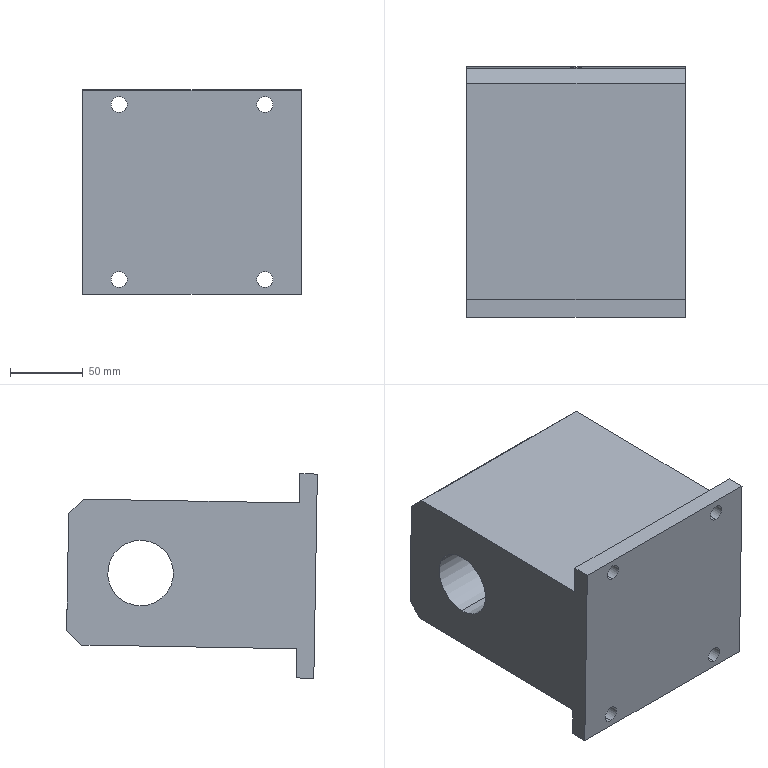Component | SolidWorks | Tailstock-1 | 1 solid | 24 faces | box 150 x 171.89 x 140.19 mm | volume 2362487 mm3 | cylinder 12 | plane 12 | commonest cylinder face diameters 11 x8 8 x2 45 x2
build123d program:
from build123d import *

# Parameters (mm, degrees)
SKETCH1_R           = 22.5
BOSS_EXTRUDE1_DEPTH = 75
CHAMFER1_SIZE       = 10
SKETCH2_R           = 5.5
CUT_EXTRUDE1_DEPTH  = 189.385
SKETCH3_R           = 4
CUT_EXTRUDE2_DEPTH  = 30


with BuildPart() as part:
    # Sketch1 → Boss-Extrude1 (new, symmetric)
    with BuildSketch(Plane.XY):
        Polygon((70, 0), (-70, 0), (-70, 12), (-50, 12), (-50, 170), (50, 170), (50, 12), (70, 12), align=None)
        with Locations((0, 120)):
            Circle(SKETCH1_R, mode=Mode.SUBTRACT)
    extrude(amount=BOSS_EXTRUDE1_DEPTH, both=True)

    # Chamfer1
    chamfer1_edges = [part.edges().sort_by_distance(p)[0] for p in [
        (-50, 170, 0),
        (50, 170, 0),
    ]]
    chamfer(chamfer1_edges, length=CHAMFER1_SIZE)

    # Sketch2 → Cut-Extrude1 (cut, through all)
    with BuildSketch(Plane(origin=(0, 12, 0), x_dir=(1, 0, 0), z_dir=(0, 1, 0))):
        with Locations(Location((-60, 50, 0), (0, 0, 180))):
            Circle(SKETCH2_R)
        with Locations((60, 50)):
            Circle(SKETCH2_R)
        with Locations(Location((60, -50, 0), (0, 0, 180))):
            Circle(SKETCH2_R)
        with Locations((-60, -50)):
            Circle(SKETCH2_R)
    extrude(amount=-CUT_EXTRUDE1_DEPTH, mode=Mode.SUBTRACT)

    # Sketch3 → Cut-Extrude2 (cut)
    with BuildSketch(Plane(origin=(0, 170, 0), x_dir=(1, 0, 0), z_dir=(0, 1, 0))):
        with Locations(Location((0, 0, 0), (0, 0, 270))):
            Circle(SKETCH3_R)
    extrude(amount=-CUT_EXTRUDE2_DEPTH, mode=Mode.SUBTRACT)


solid = part.part

# Placed as in the assembly
solid = solid.moved(Location((592.004, 1179.724, 685.022), (1, 90, 0)))
STEP:
#1=CARTESIAN_POINT('',(23.15,52.055,27.067));
#2=VERTEX_POINT('',#1);
#3=CARTESIAN_POINT('',(23.465,52.055,27.067));
#4=VERTEX_POINT('',#3);
#5=CARTESIAN_POINT('',(23.15,52.055,27.067));
#6=CARTESIAN_POINT('',(23.15,52.055,27.057));
#7=CARTESIAN_POINT('',(23.151,52.055,27.047));
#8=CARTESIAN_POINT('',(23.155,52.055,27.026));
#9=CARTESIAN_POINT('',(23.158,52.055,27.016));
#10=CARTESIAN_POINT('',(23.166,52.054,26.997));
#11=CARTESIAN_POINT('',(23.171,52.053,26.988));
#12=CARTESIAN_POINT('',(23.182,52.052,26.971));
#13=CARTESIAN_POINT('',(23.189,52.051,26.963));
#14=CARTESIAN_POINT('',(23.203,52.049,26.949));
#15=CARTESIAN_POINT('',(23.211,52.049,26.942));
#16=CARTESIAN_POINT('',(23.228,52.047,26.93));
#17=CARTESIAN_POINT('',(23.237,52.046,26.926));
#18=CARTESIAN_POINT('',(23.256,52.045,26.918));
#19=CARTESIAN_POINT('',(23.266,52.045,26.915));
#20=CARTESIAN_POINT('',(23.287,52.044,26.911));
#21=CARTESIAN_POINT('',(23.297,52.044,26.91));
#22=CARTESIAN_POINT('',(23.317,52.044,26.91));
#23=CARTESIAN_POINT('',(23.328,52.044,26.911));
#24=CARTESIAN_POINT('',(23.348,52.045,26.915));
#25=CARTESIAN_POINT('',(23.358,52.045,26.918));
#26=CARTESIAN_POINT('',(23.377,52.046,26.926));
#27=CARTESIAN_POINT('',(23.386,52.047,26.93));
#28=CARTESIAN_POINT('',(23.403,52.049,26.942));
#29=CARTESIAN_POINT('',(23.411,52.049,26.948));
#30=CARTESIAN_POINT('',(23.426,52.051,26.963));
#31=CARTESIAN_POINT('',(23.432,52.052,26.971));
#32=CARTESIAN_POINT('',(23.444,52.053,26.988));
#33=CARTESIAN_POINT('',(23.449,52.054,26.997));
#34=CARTESIAN_POINT('',(23.457,52.055,27.016));
#35=CARTESIAN_POINT('',(23.46,52.055,27.026));
#36=CARTESIAN_POINT('',(23.464,52.055,27.047));
#37=CARTESIAN_POINT('',(23.465,52.055,27.057));
#38=CARTESIAN_POINT('',(23.465,52.055,27.067));
#39=B_SPLINE_CURVE_WITH_KNOTS('',3,(#5,#6,#7,#8,#9,#10,#11,#12,#13,#14,#15,#16,#17,#18,#19,#20,#21,#22,#23,#24,#25,#26,#27,#28,#29,#30,#31,#32,#33,#34,#35,#36,#37,#38),.UNSPECIFIED.,.F.,.F.,(4,2,2,2,2,2,2,2,2,2,2,2,2,2,2,2,4),(0.,0.0007832,0.001566,0.00235,0.003133,0.003916,0.004699,0.005482,0.006265,0.007049,0.007832,0.008615,0.009398,0.01018,0.01096,0.01175,0.01253),.UNSPECIFIED.);
#40=EDGE_CURVE('',#2,#4,#39,.T.);
#41=ORIENTED_EDGE('',*,*,#40,.T.);
#42=CARTESIAN_POINT('',(23.465,53.138,27.086));
#43=VERTEX_POINT('',#42);
#44=CARTESIAN_POINT('',(23.465,51.957,27.066));
#45=DIRECTION('',(-0.,0.9998,0.01745));
#46=VECTOR('',#45,39.37);
#47=LINE('',#44,#46);
#48=EDGE_CURVE('',#4,#43,#47,.T.);
#49=ORIENTED_EDGE('',*,*,#48,.T.);
#50=CARTESIAN_POINT('',(23.15,53.138,27.086));
#51=VERTEX_POINT('',#50);
#52=CARTESIAN_POINT('',(23.307,53.138,27.086));
#53=DIRECTION('',(-0.,0.9998,0.01745));
#54=DIRECTION('',(-1.,0.,0.));
#55=AXIS2_PLACEMENT_3D('',#52,#53,#54);
#56=CIRCLE('',#55,0.1575);
#57=EDGE_CURVE('',#43,#51,#56,.T.);
#58=ORIENTED_EDGE('',*,*,#57,.T.);
#59=CARTESIAN_POINT('',(23.15,51.957,27.066));
#60=DIRECTION('',(-0.,0.9998,0.01745));
#61=VECTOR('',#60,39.37);
#62=LINE('',#59,#61);
#63=EDGE_CURVE('',#2,#51,#62,.T.);
#64=ORIENTED_EDGE('',*,*,#63,.F.);
#65=EDGE_LOOP('',(#41,#49,#58,#64));
#66=FACE_OUTER_BOUND('',#65,.T.);
#67=CARTESIAN_POINT('',(23.307,51.957,27.066));
#68=DIRECTION('',(-0.,0.9998,0.01745));
#69=DIRECTION('',(-1.,0.,0.));
#70=AXIS2_PLACEMENT_3D('',#67,#68,#69);
#71=CYLINDRICAL_SURFACE('',#70,0.1575);
#72=ADVANCED_FACE('',(#66),#71,.F.);
#73=CARTESIAN_POINT('',(21.339,46.483,24.824));
#74=VERTEX_POINT('',#73);
#75=CARTESIAN_POINT('',(21.339,46.491,24.391));
#76=VERTEX_POINT('',#75);
#77=CARTESIAN_POINT('',(21.339,46.487,24.608));
#78=DIRECTION('',(-0.,0.9998,0.01745));
#79=DIRECTION('',(0.,-0.01745,0.9998));
#80=AXIS2_PLACEMENT_3D('',#77,#78,#79);
#81=CIRCLE('',#80,0.2165);
#82=EDGE_CURVE('',#74,#76,#81,.T.);
#83=ORIENTED_EDGE('',*,*,#82,.F.);
#84=CARTESIAN_POINT('',(21.339,46.956,24.832));
#85=VERTEX_POINT('',#84);
#86=CARTESIAN_POINT('',(21.339,46.483,24.824));
#87=DIRECTION('',(-0.,0.9998,0.01745));
#88=VECTOR('',#87,39.37);
#89=LINE('',#86,#88);
#90=EDGE_CURVE('',#74,#85,#89,.T.);
#91=ORIENTED_EDGE('',*,*,#90,.T.);
#92=CARTESIAN_POINT('',(21.339,46.963,24.399));
#93=VERTEX_POINT('',#92);
#94=CARTESIAN_POINT('',(21.339,46.959,24.616));
#95=DIRECTION('',(-0.,0.9998,0.01745));
#96=DIRECTION('',(0.,-0.01745,0.9998));
#97=AXIS2_PLACEMENT_3D('',#94,#95,#96);
#98=CIRCLE('',#97,0.2165);
#99=EDGE_CURVE('',#85,#93,#98,.T.);
#100=ORIENTED_EDGE('',*,*,#99,.T.);
#101=CARTESIAN_POINT('',(21.339,46.491,24.391));
#102=DIRECTION('',(-0.,0.9998,0.01745));
#103=VECTOR('',#102,39.37);
#104=LINE('',#101,#103);
#105=EDGE_CURVE('',#76,#93,#104,.T.);
#106=ORIENTED_EDGE('',*,*,#105,.F.);
#107=EDGE_LOOP('',(#83,#91,#100,#106));
#108=FACE_OUTER_BOUND('',#107,.T.);
#109=CARTESIAN_POINT('',(21.339,46.487,24.608));
#110=DIRECTION('',(-0.,0.9998,0.01745));
#111=DIRECTION('',(0.,0.01745,-0.9998));
#112=AXIS2_PLACEMENT_3D('',#109,#110,#111);
#113=CYLINDRICAL_SURFACE('',#112,0.2165);
#114=ADVANCED_FACE('',(#108),#113,.F.);
#115=CARTESIAN_POINT('',(21.339,46.401,29.548));
#116=VERTEX_POINT('',#115);
#117=CARTESIAN_POINT('',(21.339,46.408,29.115));
#118=VERTEX_POINT('',#117);
#119=CARTESIAN_POINT('',(21.339,46.405,29.331));
#120=DIRECTION('',(-0.,0.9998,0.01745));
#121=DIRECTION('',(0.,0.01745,-0.9998));
#122=AXIS2_PLACEMENT_3D('',#119,#120,#121);
#123=CIRCLE('',#122,0.2165);
#124=EDGE_CURVE('',#116,#118,#123,.T.);
#125=ORIENTED_EDGE('',*,*,#124,.F.);
#126=CARTESIAN_POINT('',(21.339,46.873,29.556));
#127=VERTEX_POINT('',#126);
#128=CARTESIAN_POINT('',(21.339,46.401,29.548));
#129=DIRECTION('',(-0.,0.9998,0.01745));
#130=VECTOR('',#129,39.37);
#131=LINE('',#128,#130);
#132=EDGE_CURVE('',#116,#127,#131,.T.);
#133=ORIENTED_EDGE('',*,*,#132,.T.);
#134=CARTESIAN_POINT('',(21.339,46.881,29.123));
#135=VERTEX_POINT('',#134);
#136=CARTESIAN_POINT('',(21.339,46.877,29.339));
#137=DIRECTION('',(-0.,0.9998,0.01745));
#138=DIRECTION('',(0.,0.01745,-0.9998));
#139=AXIS2_PLACEMENT_3D('',#136,#137,#138);
#140=CIRCLE('',#139,0.2165);
#141=EDGE_CURVE('',#127,#135,#140,.T.);
#142=ORIENTED_EDGE('',*,*,#141,.T.);
#143=CARTESIAN_POINT('',(21.339,46.408,29.115));
#144=DIRECTION('',(-0.,0.9998,0.01745));
#145=VECTOR('',#144,39.37);
#146=LINE('',#143,#145);
#147=EDGE_CURVE('',#118,#135,#146,.T.);
#148=ORIENTED_EDGE('',*,*,#147,.F.);
#149=EDGE_LOOP('',(#125,#133,#142,#148));
#150=FACE_OUTER_BOUND('',#149,.T.);
#151=CARTESIAN_POINT('',(21.339,46.405,29.331));
#152=DIRECTION('',(-0.,0.9998,0.01745));
#153=DIRECTION('',(0.,0.01745,-0.9998));
#154=AXIS2_PLACEMENT_3D('',#151,#152,#153);
#155=CYLINDRICAL_SURFACE('',#154,0.2165);
#156=ADVANCED_FACE('',(#150),#155,.F.);
#157=CARTESIAN_POINT('',(25.276,46.401,29.548));
#158=VERTEX_POINT('',#157);
#159=CARTESIAN_POINT('',(25.276,46.408,29.115));
#160=VERTEX_POINT('',#159);
#161=CARTESIAN_POINT('',(25.276,46.405,29.331));
#162=DIRECTION('',(-0.,0.9998,0.01745));
#163=DIRECTION('',(0.,-0.01745,0.9998));
#164=AXIS2_PLACEMENT_3D('',#161,#162,#163);
#165=CIRCLE('',#164,0.2165);
#166=EDGE_CURVE('',#158,#160,#165,.T.);
#167=ORIENTED_EDGE('',*,*,#166,.F.);
#168=CARTESIAN_POINT('',(25.276,46.873,29.556));
#169=VERTEX_POINT('',#168);
#170=CARTESIAN_POINT('',(25.276,46.401,29.548));
#171=DIRECTION('',(-0.,0.9998,0.01745));
#172=VECTOR('',#171,39.37);
#173=LINE('',#170,#172);
#174=EDGE_CURVE('',#158,#169,#173,.T.);
#175=ORIENTED_EDGE('',*,*,#174,.T.);
#176=CARTESIAN_POINT('',(25.276,46.881,29.123));
#177=VERTEX_POINT('',#176);
#178=CARTESIAN_POINT('',(25.276,46.877,29.339));
#179=DIRECTION('',(-0.,0.9998,0.01745));
#180=DIRECTION('',(0.,-0.01745,0.9998));
#181=AXIS2_PLACEMENT_3D('',#178,#179,#180);
#182=CIRCLE('',#181,0.2165);
#183=EDGE_CURVE('',#169,#177,#182,.T.);
#184=ORIENTED_EDGE('',*,*,#183,.T.);
#185=CARTESIAN_POINT('',(25.276,46.408,29.115));
#186=DIRECTION('',(-0.,0.9998,0.01745));
#187=VECTOR('',#186,39.37);
#188=LINE('',#185,#187);
#189=EDGE_CURVE('',#160,#177,#188,.T.);
#190=ORIENTED_EDGE('',*,*,#189,.F.);
#191=EDGE_LOOP('',(#167,#175,#184,#190));
#192=FACE_OUTER_BOUND('',#191,.T.);
#193=CARTESIAN_POINT('',(25.276,46.405,29.331));
#194=DIRECTION('',(-0.,0.9998,0.01745));
#195=DIRECTION('',(0.,0.01745,-0.9998));
#196=AXIS2_PLACEMENT_3D('',#193,#194,#195);
#197=CYLINDRICAL_SURFACE('',#196,0.2165);
#198=ADVANCED_FACE('',(#192),#197,.F.);
#199=CARTESIAN_POINT('',(25.276,46.483,24.824));
#200=VERTEX_POINT('',#199);
#201=CARTESIAN_POINT('',(25.276,46.491,24.391));
#202=VERTEX_POINT('',#201);
#203=CARTESIAN_POINT('',(25.276,46.487,24.608));
#204=DIRECTION('',(-0.,0.9998,0.01745));
#205=DIRECTION('',(0.,0.01745,-0.9998));
#206=AXIS2_PLACEMENT_3D('',#203,#204,#205);
#207=CIRCLE('',#206,0.2165);
#208=EDGE_CURVE('',#200,#202,#207,.T.);
#209=ORIENTED_EDGE('',*,*,#208,.F.);
#210=CARTESIAN_POINT('',(25.276,46.956,24.832));
#211=VERTEX_POINT('',#210);
#212=CARTESIAN_POINT('',(25.276,46.483,24.824));
#213=DIRECTION('',(-0.,0.9998,0.01745));
#214=VECTOR('',#213,39.37);
#215=LINE('',#212,#214);
#216=EDGE_CURVE('',#200,#211,#215,.T.);
#217=ORIENTED_EDGE('',*,*,#216,.T.);
#218=CARTESIAN_POINT('',(25.276,46.963,24.399));
#219=VERTEX_POINT('',#218);
#220=CARTESIAN_POINT('',(25.276,46.959,24.616));
#221=DIRECTION('',(-0.,0.9998,0.01745));
#222=DIRECTION('',(0.,0.01745,-0.9998));
#223=AXIS2_PLACEMENT_3D('',#220,#221,#222);
#224=CIRCLE('',#223,0.2165);
#225=EDGE_CURVE('',#211,#219,#224,.T.);
#226=ORIENTED_EDGE('',*,*,#225,.T.);
#227=CARTESIAN_POINT('',(25.276,46.491,24.391));
#228=DIRECTION('',(-0.,0.9998,0.01745));
#229=VECTOR('',#228,39.37);
#230=LINE('',#227,#229);
#231=EDGE_CURVE('',#202,#219,#230,.T.);
#232=ORIENTED_EDGE('',*,*,#231,.F.);
#233=EDGE_LOOP('',(#209,#217,#226,#232));
#234=FACE_OUTER_BOUND('',#233,.T.);
#235=CARTESIAN_POINT('',(25.276,46.487,24.608));
#236=DIRECTION('',(-0.,0.9998,0.01745));
#237=DIRECTION('',(0.,0.01745,-0.9998));
#238=AXIS2_PLACEMENT_3D('',#235,#236,#237);
#239=CYLINDRICAL_SURFACE('',#238,0.2165);
#240=ADVANCED_FACE('',(#234),#239,.F.);
#241=CARTESIAN_POINT('',(20.354,51.185,26.166));
#242=VERTEX_POINT('',#241);
#243=CARTESIAN_POINT('',(20.354,51.154,27.938));
#244=VERTEX_POINT('',#243);
#245=CARTESIAN_POINT('',(20.354,51.17,27.052));
#246=DIRECTION('',(-1.,-0.,-0.));
#247=DIRECTION('',(0.,-0.01745,0.9998));
#248=AXIS2_PLACEMENT_3D('',#245,#246,#247);
#249=CIRCLE('',#248,0.8858);
#250=EDGE_CURVE('',#242,#244,#249,.T.);
#251=ORIENTED_EDGE('',*,*,#250,.T.);
#252=CARTESIAN_POINT('',(26.26,51.154,27.938));
#253=VERTEX_POINT('',#252);
#254=CARTESIAN_POINT('',(20.354,51.154,27.938));
#255=DIRECTION('',(1.,0.,0.));
#256=VECTOR('',#255,39.37);
#257=LINE('',#254,#256);
#258=EDGE_CURVE('',#244,#253,#257,.T.);
#259=ORIENTED_EDGE('',*,*,#258,.T.);
#260=CARTESIAN_POINT('',(26.26,51.185,26.166));
#261=VERTEX_POINT('',#260);
#262=CARTESIAN_POINT('',(26.26,51.17,27.052));
#263=DIRECTION('',(-1.,-0.,-0.));
#264=DIRECTION('',(0.,-0.01745,0.9998));
#265=AXIS2_PLACEMENT_3D('',#262,#263,#264);
#266=CIRCLE('',#265,0.8858);
#267=EDGE_CURVE('',#261,#253,#266,.T.);
#268=ORIENTED_EDGE('',*,*,#267,.F.);
#269=CARTESIAN_POINT('',(20.354,51.185,26.166));
#270=DIRECTION('',(1.,0.,0.));
#271=VECTOR('',#270,39.37);
#272=LINE('',#269,#271);
#273=EDGE_CURVE('',#242,#261,#272,.T.);
#274=ORIENTED_EDGE('',*,*,#273,.F.);
#275=EDGE_LOOP('',(#251,#259,#268,#274));
#276=FACE_OUTER_BOUND('',#275,.T.);
#277=CARTESIAN_POINT('',(20.354,51.17,27.052));
#278=DIRECTION('',(1.,0.,0.));
#279=DIRECTION('',(0.,0.01745,-0.9998));
#280=AXIS2_PLACEMENT_3D('',#277,#278,#279);
#281=CYLINDRICAL_SURFACE('',#280,0.8858);
#282=ADVANCED_FACE('',(#276),#281,.F.);
#283=CARTESIAN_POINT('',(20.354,53.11,28.661));
#284=VERTEX_POINT('',#283);
#285=CARTESIAN_POINT('',(20.354,53.165,25.512));
#286=VERTEX_POINT('',#285);
#287=CARTESIAN_POINT('',(20.354,53.172,25.118));
#288=DIRECTION('',(0.,0.01745,-0.9998));
#289=VECTOR('',#288,39.37);
#290=LINE('',#287,#289);
#291=EDGE_CURVE('',#284,#286,#290,.T.);
#292=ORIENTED_EDGE('',*,*,#291,.T.);
#293=CARTESIAN_POINT('',(20.354,52.778,25.111));
#294=VERTEX_POINT('',#293);
#295=CARTESIAN_POINT('',(20.354,52.778,25.111));
#296=DIRECTION('',(0.,-0.6947,-0.7193));
#297=VECTOR('',#296,39.37);
#298=LINE('',#295,#297);
#299=EDGE_CURVE('',#286,#294,#298,.T.);
#300=ORIENTED_EDGE('',*,*,#299,.T.);
#301=CARTESIAN_POINT('',(20.354,46.953,25.009));
#302=VERTEX_POINT('',#301);
#303=CARTESIAN_POINT('',(20.354,46.953,25.009));
#304=DIRECTION('',(0.,-0.9998,-0.01745));
#305=VECTOR('',#304,39.37);
#306=LINE('',#303,#305);
#307=EDGE_CURVE('',#294,#302,#306,.T.);
#308=ORIENTED_EDGE('',*,*,#307,.T.);
#309=CARTESIAN_POINT('',(20.354,46.966,24.222));
#310=VERTEX_POINT('',#309);
#311=CARTESIAN_POINT('',(20.354,46.966,24.222));
#312=DIRECTION('',(-0.,0.01745,-0.9998));
#313=VECTOR('',#312,39.37);
#314=LINE('',#311,#313);
#315=EDGE_CURVE('',#302,#310,#314,.T.);
#316=ORIENTED_EDGE('',*,*,#315,.T.);
#317=CARTESIAN_POINT('',(20.354,46.494,24.214));
#318=VERTEX_POINT('',#317);
#319=CARTESIAN_POINT('',(20.354,46.494,24.214));
#320=DIRECTION('',(0.,-0.9998,-0.01745));
#321=VECTOR('',#320,39.37);
#322=LINE('',#319,#321);
#323=EDGE_CURVE('',#310,#318,#322,.T.);
#324=ORIENTED_EDGE('',*,*,#323,.T.);
#325=CARTESIAN_POINT('',(20.354,46.398,29.725));
#326=VERTEX_POINT('',#325);
#327=CARTESIAN_POINT('',(20.354,46.398,29.725));
#328=DIRECTION('',(0.,-0.01745,0.9998));
#329=VECTOR('',#328,39.37);
#330=LINE('',#327,#329);
#331=EDGE_CURVE('',#318,#326,#330,.T.);
#332=ORIENTED_EDGE('',*,*,#331,.T.);
#333=CARTESIAN_POINT('',(20.354,46.87,29.733));
#334=VERTEX_POINT('',#333);
#335=CARTESIAN_POINT('',(20.354,46.398,29.725));
#336=DIRECTION('',(-0.,0.9998,0.01745));
#337=VECTOR('',#336,39.37);
#338=LINE('',#335,#337);
#339=EDGE_CURVE('',#326,#334,#338,.T.);
#340=ORIENTED_EDGE('',*,*,#339,.T.);
#341=CARTESIAN_POINT('',(20.354,46.884,28.946));
#342=VERTEX_POINT('',#341);
#343=CARTESIAN_POINT('',(20.354,46.87,29.733));
#344=DIRECTION('',(0.,0.01745,-0.9998));
#345=VECTOR('',#344,39.37);
#346=LINE('',#343,#345);
#347=EDGE_CURVE('',#334,#342,#346,.T.);
#348=ORIENTED_EDGE('',*,*,#347,.T.);
#349=CARTESIAN_POINT('',(20.354,52.71,29.047));
#350=VERTEX_POINT('',#349);
#351=CARTESIAN_POINT('',(20.354,46.884,28.946));
#352=DIRECTION('',(-0.,0.9998,0.01745));
#353=VECTOR('',#352,39.37);
#354=LINE('',#351,#353);
#355=EDGE_CURVE('',#342,#350,#354,.T.);
#356=ORIENTED_EDGE('',*,*,#355,.T.);
#357=CARTESIAN_POINT('',(20.354,53.11,28.661));
#358=DIRECTION('',(-0.,0.7193,-0.6947));
#359=VECTOR('',#358,39.37);
#360=LINE('',#357,#359);
#361=EDGE_CURVE('',#350,#284,#360,.T.);
#362=ORIENTED_EDGE('',*,*,#361,.T.);
#363=EDGE_LOOP('',(#292,#300,#308,#316,#324,#332,#340,#348,#356,#362));
#364=FACE_OUTER_BOUND('',#363,.T.);
#365=ORIENTED_EDGE('',*,*,#250,.F.);
#366=CARTESIAN_POINT('',(20.354,51.17,27.052));
#367=DIRECTION('',(-1.,-0.,-0.));
#368=DIRECTION('',(0.,-0.01745,0.9998));
#369=AXIS2_PLACEMENT_3D('',#366,#367,#368);
#370=CIRCLE('',#369,0.8858);
#371=EDGE_CURVE('',#244,#242,#370,.T.);
#372=ORIENTED_EDGE('',*,*,#371,.F.);
#373=EDGE_LOOP('',(#365,#372));
#374=FACE_BOUND('',#373,.T.);
#375=CARTESIAN_POINT('',(20.354,46.446,26.969));
#376=DIRECTION('',(1.,0.,0.));
#377=DIRECTION('',(0.,0.01745,-0.9998));
#378=AXIS2_PLACEMENT_3D('',#375,#376,#377);
#379=PLANE('',#378);
#380=ADVANCED_FACE('',(#364,#374),#379,.F.);
#381=CARTESIAN_POINT('',(26.26,52.778,25.111));
#382=VERTEX_POINT('',#381);
#383=CARTESIAN_POINT('',(26.26,46.953,25.009));
#384=VERTEX_POINT('',#383);
#385=CARTESIAN_POINT('',(26.26,46.953,25.009));
#386=DIRECTION('',(0.,-0.9998,-0.01745));
#387=VECTOR('',#386,39.37);
#388=LINE('',#385,#387);
#389=EDGE_CURVE('',#382,#384,#388,.T.);
#390=ORIENTED_EDGE('',*,*,#389,.F.);
#391=CARTESIAN_POINT('',(26.26,53.165,25.512));
#392=VERTEX_POINT('',#391);
#393=CARTESIAN_POINT('',(26.26,50.651,22.908));
#394=DIRECTION('',(-0.,0.6947,0.7193));
#395=VECTOR('',#394,39.37);
#396=LINE('',#393,#395);
#397=EDGE_CURVE('',#382,#392,#396,.T.);
#398=ORIENTED_EDGE('',*,*,#397,.T.);
#399=CARTESIAN_POINT('',(26.26,53.11,28.661));
#400=VERTEX_POINT('',#399);
#401=CARTESIAN_POINT('',(26.26,53.172,25.118));
#402=DIRECTION('',(0.,0.01745,-0.9998));
#403=VECTOR('',#402,39.37);
#404=LINE('',#401,#403);
#405=EDGE_CURVE('',#400,#392,#404,.T.);
#406=ORIENTED_EDGE('',*,*,#405,.F.);
#407=CARTESIAN_POINT('',(26.26,52.71,29.047));
#408=VERTEX_POINT('',#407);
#409=CARTESIAN_POINT('',(26.26,50.507,31.175));
#410=DIRECTION('',(0.,-0.7193,0.6947));
#411=VECTOR('',#410,39.37);
#412=LINE('',#409,#411);
#413=EDGE_CURVE('',#400,#408,#412,.T.);
#414=ORIENTED_EDGE('',*,*,#413,.T.);
#415=CARTESIAN_POINT('',(26.26,46.884,28.946));
#416=VERTEX_POINT('',#415);
#417=CARTESIAN_POINT('',(26.26,46.884,28.946));
#418=DIRECTION('',(-0.,0.9998,0.01745));
#419=VECTOR('',#418,39.37);
#420=LINE('',#417,#419);
#421=EDGE_CURVE('',#416,#408,#420,.T.);
#422=ORIENTED_EDGE('',*,*,#421,.F.);
#423=CARTESIAN_POINT('',(26.26,46.87,29.733));
#424=VERTEX_POINT('',#423);
#425=CARTESIAN_POINT('',(26.26,46.87,29.733));
#426=DIRECTION('',(0.,0.01745,-0.9998));
#427=VECTOR('',#426,39.37);
#428=LINE('',#425,#427);
#429=EDGE_CURVE('',#424,#416,#428,.T.);
#430=ORIENTED_EDGE('',*,*,#429,.F.);
#431=CARTESIAN_POINT('',(26.26,46.398,29.725));
#432=VERTEX_POINT('',#431);
#433=CARTESIAN_POINT('',(26.26,46.398,29.725));
#434=DIRECTION('',(-0.,0.9998,0.01745));
#435=VECTOR('',#434,39.37);
#436=LINE('',#433,#435);
#437=EDGE_CURVE('',#432,#424,#436,.T.);
#438=ORIENTED_EDGE('',*,*,#437,.F.);
#439=CARTESIAN_POINT('',(26.26,46.494,24.214));
#440=VERTEX_POINT('',#439);
#441=CARTESIAN_POINT('',(26.26,46.398,29.725));
#442=DIRECTION('',(0.,-0.01745,0.9998));
#443=VECTOR('',#442,39.37);
#444=LINE('',#441,#443);
#445=EDGE_CURVE('',#440,#432,#444,.T.);
#446=ORIENTED_EDGE('',*,*,#445,.F.);
#447=CARTESIAN_POINT('',(26.26,46.966,24.222));
#448=VERTEX_POINT('',#447);
#449=CARTESIAN_POINT('',(26.26,46.494,24.214));
#450=DIRECTION('',(0.,-0.9998,-0.01745));
#451=VECTOR('',#450,39.37);
#452=LINE('',#449,#451);
#453=EDGE_CURVE('',#448,#440,#452,.T.);
#454=ORIENTED_EDGE('',*,*,#453,.F.);
#455=CARTESIAN_POINT('',(26.26,46.966,24.222));
#456=DIRECTION('',(-0.,0.01745,-0.9998));
#457=VECTOR('',#456,39.37);
#458=LINE('',#455,#457);
#459=EDGE_CURVE('',#384,#448,#458,.T.);
#460=ORIENTED_EDGE('',*,*,#459,.F.);
#461=EDGE_LOOP('',(#390,#398,#406,#414,#422,#430,#438,#446,#454,#460));
#462=FACE_OUTER_BOUND('',#461,.T.);
#463=ORIENTED_EDGE('',*,*,#267,.T.);
#464=CARTESIAN_POINT('',(26.26,51.17,27.052));
#465=DIRECTION('',(-1.,-0.,-0.));
#466=DIRECTION('',(0.,-0.01745,0.9998));
#467=AXIS2_PLACEMENT_3D('',#464,#465,#466);
#468=CIRCLE('',#467,0.8858);
#469=EDGE_CURVE('',#253,#261,#468,.T.);
#470=ORIENTED_EDGE('',*,*,#469,.T.);
#471=EDGE_LOOP('',(#463,#470));
#472=FACE_BOUND('',#471,.T.);
#473=CARTESIAN_POINT('',(26.26,46.446,26.969));
#474=DIRECTION('',(1.,0.,0.));
#475=DIRECTION('',(0.,0.01745,-0.9998));
#476=AXIS2_PLACEMENT_3D('',#473,#474,#475);
#477=PLANE('',#476);
#478=ADVANCED_FACE('',(#462,#472),#477,.T.);
#479=ORIENTED_EDGE('',*,*,#453,.T.);
#480=CARTESIAN_POINT('',(20.354,46.494,24.214));
#481=DIRECTION('',(1.,0.,0.));
#482=VECTOR('',#481,39.37);
#483=LINE('',#480,#482);
#484=EDGE_CURVE('',#318,#440,#483,.T.);
#485=ORIENTED_EDGE('',*,*,#484,.F.);
#486=ORIENTED_EDGE('',*,*,#323,.F.);
#487=CARTESIAN_POINT('',(20.354,46.966,24.222));
#488=DIRECTION('',(1.,0.,0.));
#489=VECTOR('',#488,39.37);
#490=LINE('',#487,#489);
#491=EDGE_CURVE('',#310,#448,#490,.T.);
#492=ORIENTED_EDGE('',*,*,#491,.T.);
#493=EDGE_LOOP('',(#479,#485,#486,#492));
#494=FACE_OUTER_BOUND('',#493,.T.);
#495=CARTESIAN_POINT('',(20.354,46.494,24.214));
#496=DIRECTION('',(0.,-0.01745,0.9998));
#497=DIRECTION('',(1.,0.,0.));
#498=AXIS2_PLACEMENT_3D('',#495,#496,#497);
#499=PLANE('',#498);
#500=ADVANCED_FACE('',(#494),#499,.F.);
#501=CARTESIAN_POINT('',(21.339,46.487,24.608));
#502=DIRECTION('',(-0.,0.9998,0.01745));
#503=DIRECTION('',(0.,-0.01745,0.9998));
#504=AXIS2_PLACEMENT_3D('',#501,#502,#503);
#505=CIRCLE('',#504,0.2165);
#506=EDGE_CURVE('',#76,#74,#505,.T.);
#507=ORIENTED_EDGE('',*,*,#506,.T.);
#508=ORIENTED_EDGE('',*,*,#82,.T.);
#509=EDGE_LOOP('',(#507,#508));
#510=FACE_BOUND('',#509,.T.);
#511=CARTESIAN_POINT('',(21.339,46.405,29.331));
#512=DIRECTION('',(-0.,0.9998,0.01745));
#513=DIRECTION('',(0.,0.01745,-0.9998));
#514=AXIS2_PLACEMENT_3D('',#511,#512,#513);
#515=CIRCLE('',#514,0.2165);
#516=EDGE_CURVE('',#118,#116,#515,.T.);
#517=ORIENTED_EDGE('',*,*,#516,.T.);
#518=ORIENTED_EDGE('',*,*,#124,.T.);
#519=EDGE_LOOP('',(#517,#518));
#520=FACE_BOUND('',#519,.T.);
#521=CARTESIAN_POINT('',(25.276,46.405,29.331));
#522=DIRECTION('',(-0.,0.9998,0.01745));
#523=DIRECTION('',(0.,-0.01745,0.9998));
#524=AXIS2_PLACEMENT_3D('',#521,#522,#523);
#525=CIRCLE('',#524,0.2165);
#526=EDGE_CURVE('',#160,#158,#525,.T.);
#527=ORIENTED_EDGE('',*,*,#526,.T.);
#528=ORIENTED_EDGE('',*,*,#166,.T.);
#529=EDGE_LOOP('',(#527,#528));
#530=FACE_BOUND('',#529,.T.);
#531=CARTESIAN_POINT('',(25.276,46.487,24.608));
#532=DIRECTION('',(-0.,0.9998,0.01745));
#533=DIRECTION('',(0.,0.01745,-0.9998));
#534=AXIS2_PLACEMENT_3D('',#531,#532,#533);
#535=CIRCLE('',#534,0.2165);
#536=EDGE_CURVE('',#202,#200,#535,.T.);
#537=ORIENTED_EDGE('',*,*,#536,.T.);
#538=ORIENTED_EDGE('',*,*,#208,.T.);
#539=EDGE_LOOP('',(#537,#538));
#540=FACE_BOUND('',#539,.T.);
#541=ORIENTED_EDGE('',*,*,#445,.T.);
#542=CARTESIAN_POINT('',(20.354,46.398,29.725));
#543=DIRECTION('',(1.,0.,0.));
#544=VECTOR('',#543,39.37);
#545=LINE('',#542,#544);
#546=EDGE_CURVE('',#326,#432,#545,.T.);
#547=ORIENTED_EDGE('',*,*,#546,.F.);
#548=ORIENTED_EDGE('',*,*,#331,.F.);
#549=ORIENTED_EDGE('',*,*,#484,.T.);
#550=EDGE_LOOP('',(#541,#547,#548,#549));
#551=FACE_OUTER_BOUND('',#550,.T.);
#552=CARTESIAN_POINT('',(20.354,46.398,29.725));
#553=DIRECTION('',(-0.,0.9998,0.01745));
#554=DIRECTION('',(-1.,-0.,-0.));
#555=AXIS2_PLACEMENT_3D('',#552,#553,#554);
#556=PLANE('',#555);
#557=ADVANCED_FACE('',(#510,#520,#530,#540,#551),#556,.F.);
#558=ORIENTED_EDGE('',*,*,#437,.T.);
#559=CARTESIAN_POINT('',(20.354,46.87,29.733));
#560=DIRECTION('',(1.,0.,0.));
#561=VECTOR('',#560,39.37);
#562=LINE('',#559,#561);
#563=EDGE_CURVE('',#334,#424,#562,.T.);
#564=ORIENTED_EDGE('',*,*,#563,.F.);
#565=ORIENTED_EDGE('',*,*,#339,.F.);
#566=ORIENTED_EDGE('',*,*,#546,.T.);
#567=EDGE_LOOP('',(#558,#564,#565,#566));
#568=FACE_OUTER_BOUND('',#567,.T.);
#569=CARTESIAN_POINT('',(20.354,46.398,29.725));
#570=DIRECTION('',(0.,0.01745,-0.9998));
#571=DIRECTION('',(-1.,-0.,-0.));
#572=AXIS2_PLACEMENT_3D('',#569,#570,#571);
#573=PLANE('',#572);
#574=ADVANCED_FACE('',(#568),#573,.F.);
#575=CARTESIAN_POINT('',(21.339,46.877,29.339));
#576=DIRECTION('',(-0.,0.9998,0.01745));
#577=DIRECTION('',(0.,0.01745,-0.9998));
#578=AXIS2_PLACEMENT_3D('',#575,#576,#577);
#579=CIRCLE('',#578,0.2165);
#580=EDGE_CURVE('',#135,#127,#579,.T.);
#581=ORIENTED_EDGE('',*,*,#580,.F.);
#582=ORIENTED_EDGE('',*,*,#141,.F.);
#583=EDGE_LOOP('',(#581,#582));
#584=FACE_BOUND('',#583,.T.);
#585=CARTESIAN_POINT('',(25.276,46.877,29.339));
#586=DIRECTION('',(-0.,0.9998,0.01745));
#587=DIRECTION('',(0.,-0.01745,0.9998));
#588=AXIS2_PLACEMENT_3D('',#585,#586,#587);
#589=CIRCLE('',#588,0.2165);
#590=EDGE_CURVE('',#177,#169,#589,.T.);
#591=ORIENTED_EDGE('',*,*,#590,.F.);
#592=ORIENTED_EDGE('',*,*,#183,.F.);
#593=EDGE_LOOP('',(#591,#592));
#594=FACE_BOUND('',#593,.T.);
#595=ORIENTED_EDGE('',*,*,#429,.T.);
#596=CARTESIAN_POINT('',(20.354,46.884,28.946));
#597=DIRECTION('',(1.,0.,0.));
#598=VECTOR('',#597,39.37);
#599=LINE('',#596,#598);
#600=EDGE_CURVE('',#342,#416,#599,.T.);
#601=ORIENTED_EDGE('',*,*,#600,.F.);
#602=ORIENTED_EDGE('',*,*,#347,.F.);
#603=ORIENTED_EDGE('',*,*,#563,.T.);
#604=EDGE_LOOP('',(#595,#601,#602,#603));
#605=FACE_OUTER_BOUND('',#604,.T.);
#606=CARTESIAN_POINT('',(20.354,46.87,29.733));
#607=DIRECTION('',(0.,-0.9998,-0.01745));
#608=DIRECTION('',(-0.,-0.01745,0.9998));
#609=AXIS2_PLACEMENT_3D('',#606,#607,#608);
#610=PLANE('',#609);
#611=ADVANCED_FACE('',(#584,#594,#605),#610,.F.);
#612=ORIENTED_EDGE('',*,*,#421,.T.);
#613=CARTESIAN_POINT('',(20.354,52.71,29.047));
#614=DIRECTION('',(-1.,-0.,-0.));
#615=VECTOR('',#614,39.37);
#616=LINE('',#613,#615);
#617=EDGE_CURVE('',#408,#350,#616,.T.);
#618=ORIENTED_EDGE('',*,*,#617,.T.);
#619=ORIENTED_EDGE('',*,*,#355,.F.);
#620=ORIENTED_EDGE('',*,*,#600,.T.);
#621=EDGE_LOOP('',(#612,#618,#619,#620));
#622=FACE_OUTER_BOUND('',#621,.T.);
#623=CARTESIAN_POINT('',(20.354,46.884,28.946));
#624=DIRECTION('',(0.,0.01745,-0.9998));
#625=DIRECTION('',(-1.,-0.,-0.));
#626=AXIS2_PLACEMENT_3D('',#623,#624,#625);
#627=PLANE('',#626);
#628=ADVANCED_FACE('',(#622),#627,.F.);
#629=CARTESIAN_POINT('',(23.307,53.138,27.086));
#630=DIRECTION('',(-0.,0.9998,0.01745));
#631=DIRECTION('',(-1.,0.,0.));
#632=AXIS2_PLACEMENT_3D('',#629,#630,#631);
#633=CIRCLE('',#632,0.1575);
#634=EDGE_CURVE('',#51,#43,#633,.T.);
#635=ORIENTED_EDGE('',*,*,#634,.F.);
#636=ORIENTED_EDGE('',*,*,#57,.F.);
#637=EDGE_LOOP('',(#635,#636));
#638=FACE_BOUND('',#637,.T.);
#639=ORIENTED_EDGE('',*,*,#405,.T.);
#640=CARTESIAN_POINT('',(20.354,53.165,25.512));
#641=DIRECTION('',(-1.,-0.,-0.));
#642=VECTOR('',#641,39.37);
#643=LINE('',#640,#642);
#644=EDGE_CURVE('',#392,#286,#643,.T.);
#645=ORIENTED_EDGE('',*,*,#644,.T.);
#646=ORIENTED_EDGE('',*,*,#291,.F.);
#647=CARTESIAN_POINT('',(20.354,53.11,28.661));
#648=DIRECTION('',(1.,0.,0.));
#649=VECTOR('',#648,39.37);
#650=LINE('',#647,#649);
#651=EDGE_CURVE('',#284,#400,#650,.T.);
#652=ORIENTED_EDGE('',*,*,#651,.T.);
#653=EDGE_LOOP('',(#639,#645,#646,#652));
#654=FACE_OUTER_BOUND('',#653,.T.);
#655=CARTESIAN_POINT('',(20.354,53.172,25.118));
#656=DIRECTION('',(0.,-0.9998,-0.01745));
#657=DIRECTION('',(1.,0.,0.));
#658=AXIS2_PLACEMENT_3D('',#655,#656,#657);
#659=PLANE('',#658);
#660=ADVANCED_FACE('',(#638,#654),#659,.F.);
#661=ORIENTED_EDGE('',*,*,#307,.F.);
#662=CARTESIAN_POINT('',(20.354,52.778,25.111));
#663=DIRECTION('',(1.,0.,0.));
#664=VECTOR('',#663,39.37);
#665=LINE('',#662,#664);
#666=EDGE_CURVE('',#294,#382,#665,.T.);
#667=ORIENTED_EDGE('',*,*,#666,.T.);
#668=ORIENTED_EDGE('',*,*,#389,.T.);
#669=CARTESIAN_POINT('',(20.354,46.953,25.009));
#670=DIRECTION('',(1.,0.,0.));
#671=VECTOR('',#670,39.37);
#672=LINE('',#669,#671);
#673=EDGE_CURVE('',#302,#384,#672,.T.);
#674=ORIENTED_EDGE('',*,*,#673,.F.);
#675=EDGE_LOOP('',(#661,#667,#668,#674));
#676=FACE_OUTER_BOUND('',#675,.T.);
#677=CARTESIAN_POINT('',(20.354,46.953,25.009));
#678=DIRECTION('',(0.,-0.01745,0.9998));
#679=DIRECTION('',(1.,0.,0.));
#680=AXIS2_PLACEMENT_3D('',#677,#678,#679);
#681=PLANE('',#680);
#682=ADVANCED_FACE('',(#676),#681,.F.);
#683=CARTESIAN_POINT('',(21.339,46.959,24.616));
#684=DIRECTION('',(-0.,0.9998,0.01745));
#685=DIRECTION('',(0.,-0.01745,0.9998));
#686=AXIS2_PLACEMENT_3D('',#683,#684,#685);
#687=CIRCLE('',#686,0.2165);
#688=EDGE_CURVE('',#93,#85,#687,.T.);
#689=ORIENTED_EDGE('',*,*,#688,.F.);
#690=ORIENTED_EDGE('',*,*,#99,.F.);
#691=EDGE_LOOP('',(#689,#690));
#692=FACE_BOUND('',#691,.T.);
#693=CARTESIAN_POINT('',(25.276,46.959,24.616));
#694=DIRECTION('',(-0.,0.9998,0.01745));
#695=DIRECTION('',(0.,0.01745,-0.9998));
#696=AXIS2_PLACEMENT_3D('',#693,#694,#695);
#697=CIRCLE('',#696,0.2165);
#698=EDGE_CURVE('',#219,#211,#697,.T.);
#699=ORIENTED_EDGE('',*,*,#698,.F.);
#700=ORIENTED_EDGE('',*,*,#225,.F.);
#701=EDGE_LOOP('',(#699,#700));
#702=FACE_BOUND('',#701,.T.);
#703=ORIENTED_EDGE('',*,*,#459,.T.);
#704=ORIENTED_EDGE('',*,*,#491,.F.);
#705=ORIENTED_EDGE('',*,*,#315,.F.);
#706=ORIENTED_EDGE('',*,*,#673,.T.);
#707=EDGE_LOOP('',(#703,#704,#705,#706));
#708=FACE_OUTER_BOUND('',#707,.T.);
#709=CARTESIAN_POINT('',(20.354,46.966,24.222));
#710=DIRECTION('',(0.,-0.9998,-0.01745));
#711=DIRECTION('',(0.,-0.01745,0.9998));
#712=AXIS2_PLACEMENT_3D('',#709,#710,#711);
#713=PLANE('',#712);
#714=ADVANCED_FACE('',(#692,#702,#708),#713,.F.);
#715=ORIENTED_EDGE('',*,*,#258,.F.);
#716=ORIENTED_EDGE('',*,*,#371,.T.);
#717=ORIENTED_EDGE('',*,*,#273,.T.);
#718=ORIENTED_EDGE('',*,*,#469,.F.);
#719=EDGE_LOOP('',(#715,#716,#717,#718));
#720=FACE_OUTER_BOUND('',#719,.T.);
#721=ORIENTED_EDGE('',*,*,#40,.F.);
#722=CARTESIAN_POINT('',(23.465,52.055,27.067));
#723=CARTESIAN_POINT('',(23.465,52.055,27.078));
#724=CARTESIAN_POINT('',(23.464,52.055,27.088));
#725=CARTESIAN_POINT('',(23.46,52.054,27.108));
#726=CARTESIAN_POINT('',(23.457,52.053,27.118));
#727=CARTESIAN_POINT('',(23.449,52.051,27.137));
#728=CARTESIAN_POINT('',(23.444,52.05,27.146));
#729=CARTESIAN_POINT('',(23.432,52.048,27.163));
#730=CARTESIAN_POINT('',(23.426,52.047,27.171));
#731=CARTESIAN_POINT('',(23.411,52.045,27.186));
#732=CARTESIAN_POINT('',(23.403,52.044,27.192));
#733=CARTESIAN_POINT('',(23.386,52.042,27.204));
#734=CARTESIAN_POINT('',(23.377,52.041,27.208));
#735=CARTESIAN_POINT('',(23.358,52.04,27.216));
#736=CARTESIAN_POINT('',(23.348,52.039,27.219));
#737=CARTESIAN_POINT('',(23.328,52.039,27.223));
#738=CARTESIAN_POINT('',(23.318,52.038,27.224));
#739=CARTESIAN_POINT('',(23.297,52.038,27.224));
#740=CARTESIAN_POINT('',(23.287,52.039,27.223));
#741=CARTESIAN_POINT('',(23.267,52.039,27.219));
#742=CARTESIAN_POINT('',(23.256,52.04,27.216));
#743=CARTESIAN_POINT('',(23.237,52.041,27.209));
#744=CARTESIAN_POINT('',(23.228,52.042,27.204));
#745=CARTESIAN_POINT('',(23.211,52.044,27.192));
#746=CARTESIAN_POINT('',(23.203,52.045,27.186));
#747=CARTESIAN_POINT('',(23.189,52.047,27.171));
#748=CARTESIAN_POINT('',(23.182,52.048,27.163));
#749=CARTESIAN_POINT('',(23.171,52.05,27.146));
#750=CARTESIAN_POINT('',(23.166,52.051,27.137));
#751=CARTESIAN_POINT('',(23.158,52.053,27.118));
#752=CARTESIAN_POINT('',(23.155,52.054,27.108));
#753=CARTESIAN_POINT('',(23.151,52.055,27.088));
#754=CARTESIAN_POINT('',(23.15,52.055,27.078));
#755=CARTESIAN_POINT('',(23.15,52.055,27.067));
#756=B_SPLINE_CURVE_WITH_KNOTS('',3,(#722,#723,#724,#725,#726,#727,#728,#729,#730,#731,#732,#733,#734,#735,#736,#737,#738,#739,#740,#741,#742,#743,#744,#745,#746,#747,#748,#749,#750,#751,#752,#753,#754,#755),.UNSPECIFIED.,.F.,.F.,(4,2,2,2,2,2,2,2,2,2,2,2,2,2,2,2,4),(0.01253,0.01331,0.0141,0.01488,0.01566,0.01645,0.01723,0.01801,0.01879,0.01958,0.02036,0.02114,0.02193,0.02271,0.02349,0.02428,0.02506),.UNSPECIFIED.);
#757=EDGE_CURVE('',#4,#2,#756,.T.);
#758=ORIENTED_EDGE('',*,*,#757,.F.);
#759=EDGE_LOOP('',(#721,#758));
#760=FACE_BOUND('',#759,.T.);
#761=CARTESIAN_POINT('',(20.354,51.17,27.052));
#762=DIRECTION('',(1.,0.,0.));
#763=DIRECTION('',(0.,0.01745,-0.9998));
#764=AXIS2_PLACEMENT_3D('',#761,#762,#763);
#765=CYLINDRICAL_SURFACE('',#764,0.8858);
#766=ADVANCED_FACE('',(#720,#760),#765,.F.);
#767=ORIENTED_EDGE('',*,*,#299,.F.);
#768=ORIENTED_EDGE('',*,*,#644,.F.);
#769=ORIENTED_EDGE('',*,*,#397,.F.);
#770=ORIENTED_EDGE('',*,*,#666,.F.);
#771=EDGE_LOOP('',(#767,#768,#769,#770));
#772=FACE_OUTER_BOUND('',#771,.T.);
#773=CARTESIAN_POINT('',(20.354,52.778,25.111));
#774=DIRECTION('',(0.,-0.7193,0.6947));
#775=DIRECTION('',(1.,0.,0.));
#776=AXIS2_PLACEMENT_3D('',#773,#774,#775);
#777=PLANE('',#776);
#778=ADVANCED_FACE('',(#772),#777,.F.);
#779=ORIENTED_EDGE('',*,*,#361,.F.);
#780=ORIENTED_EDGE('',*,*,#617,.F.);
#781=ORIENTED_EDGE('',*,*,#413,.F.);
#782=ORIENTED_EDGE('',*,*,#651,.F.);
#783=EDGE_LOOP('',(#779,#780,#781,#782));
#784=FACE_OUTER_BOUND('',#783,.T.);
#785=CARTESIAN_POINT('',(20.354,53.11,28.661));
#786=DIRECTION('',(0.,-0.6947,-0.7193));
#787=DIRECTION('',(1.,0.,0.));
#788=AXIS2_PLACEMENT_3D('',#785,#786,#787);
#789=PLANE('',#788);
#790=ADVANCED_FACE('',(#784),#789,.F.);
#791=ORIENTED_EDGE('',*,*,#216,.F.);
#792=ORIENTED_EDGE('',*,*,#536,.F.);
#793=ORIENTED_EDGE('',*,*,#231,.T.);
#794=ORIENTED_EDGE('',*,*,#698,.T.);
#795=EDGE_LOOP('',(#791,#792,#793,#794));
#796=FACE_OUTER_BOUND('',#795,.T.);
#797=CARTESIAN_POINT('',(25.276,46.487,24.608));
#798=DIRECTION('',(-0.,0.9998,0.01745));
#799=DIRECTION('',(0.,0.01745,-0.9998));
#800=AXIS2_PLACEMENT_3D('',#797,#798,#799);
#801=CYLINDRICAL_SURFACE('',#800,0.2165);
#802=ADVANCED_FACE('',(#796),#801,.F.);
#803=ORIENTED_EDGE('',*,*,#174,.F.);
#804=ORIENTED_EDGE('',*,*,#526,.F.);
#805=ORIENTED_EDGE('',*,*,#189,.T.);
#806=ORIENTED_EDGE('',*,*,#590,.T.);
#807=EDGE_LOOP('',(#803,#804,#805,#806));
#808=FACE_OUTER_BOUND('',#807,.T.);
#809=CARTESIAN_POINT('',(25.276,46.405,29.331));
#810=DIRECTION('',(-0.,0.9998,0.01745));
#811=DIRECTION('',(0.,0.01745,-0.9998));
#812=AXIS2_PLACEMENT_3D('',#809,#810,#811);
#813=CYLINDRICAL_SURFACE('',#812,0.2165);
#814=ADVANCED_FACE('',(#808),#813,.F.);
#815=ORIENTED_EDGE('',*,*,#132,.F.);
#816=ORIENTED_EDGE('',*,*,#516,.F.);
#817=ORIENTED_EDGE('',*,*,#147,.T.);
#818=ORIENTED_EDGE('',*,*,#580,.T.);
#819=EDGE_LOOP('',(#815,#816,#817,#818));
#820=FACE_OUTER_BOUND('',#819,.T.);
#821=CARTESIAN_POINT('',(21.339,46.405,29.331));
#822=DIRECTION('',(-0.,0.9998,0.01745));
#823=DIRECTION('',(0.,0.01745,-0.9998));
#824=AXIS2_PLACEMENT_3D('',#821,#822,#823);
#825=CYLINDRICAL_SURFACE('',#824,0.2165);
#826=ADVANCED_FACE('',(#820),#825,.F.);
#827=ORIENTED_EDGE('',*,*,#90,.F.);
#828=ORIENTED_EDGE('',*,*,#506,.F.);
#829=ORIENTED_EDGE('',*,*,#105,.T.);
#830=ORIENTED_EDGE('',*,*,#688,.T.);
#831=EDGE_LOOP('',(#827,#828,#829,#830));
#832=FACE_OUTER_BOUND('',#831,.T.);
#833=CARTESIAN_POINT('',(21.339,46.487,24.608));
#834=DIRECTION('',(-0.,0.9998,0.01745));
#835=DIRECTION('',(0.,0.01745,-0.9998));
#836=AXIS2_PLACEMENT_3D('',#833,#834,#835);
#837=CYLINDRICAL_SURFACE('',#836,0.2165);
#838=ADVANCED_FACE('',(#832),#837,.F.);
#839=ORIENTED_EDGE('',*,*,#48,.F.);
#840=ORIENTED_EDGE('',*,*,#757,.T.);
#841=ORIENTED_EDGE('',*,*,#63,.T.);
#842=ORIENTED_EDGE('',*,*,#634,.T.);
#843=EDGE_LOOP('',(#839,#840,#841,#842));
#844=FACE_OUTER_BOUND('',#843,.T.);
#845=CARTESIAN_POINT('',(23.307,51.957,27.066));
#846=DIRECTION('',(-0.,0.9998,0.01745));
#847=DIRECTION('',(-1.,0.,0.));
#848=AXIS2_PLACEMENT_3D('',#845,#846,#847);
#849=CYLINDRICAL_SURFACE('',#848,0.1575);
#850=ADVANCED_FACE('',(#844),#849,.F.);
#851=CLOSED_SHELL('',(#72,#114,#156,#198,#240,#282,#380,#478,#500,#557,#574,#611,#628,#660,#682,#714,#766,#778,#790,#802,#814,#826,#838,#850));
#852=MANIFOLD_SOLID_BREP('',#851);
#853=CARTESIAN_POINT('',(0.,0.,0.));
#854=DIRECTION('',(0.,0.,1.));
#855=DIRECTION('',(1.,0.,0.));
#856=AXIS2_PLACEMENT_3D('',#853,#854,#855);
#857=(LENGTH_UNIT()NAMED_UNIT(*)SI_UNIT($,.METRE.));
#858=LENGTH_MEASURE_WITH_UNIT(LENGTH_MEASURE(0.0254),#857);
#859=DIMENSIONAL_EXPONENTS(1.,0.,0.,0.,0.,0.,0.);
#860=(CONVERSION_BASED_UNIT('',#858)LENGTH_UNIT()NAMED_UNIT(#859));
#861=UNCERTAINTY_MEASURE_WITH_UNIT(LENGTH_MEASURE(0.00001),#860,'','');
#862=(NAMED_UNIT(*)PLANE_ANGLE_UNIT()SI_UNIT($,.RADIAN.));
#863=(NAMED_UNIT(*)SI_UNIT($,.STERADIAN.)SOLID_ANGLE_UNIT());
#864=(GEOMETRIC_REPRESENTATION_CONTEXT(3)GLOBAL_UNCERTAINTY_ASSIGNED_CONTEXT((#861))GLOBAL_UNIT_ASSIGNED_CONTEXT((#860,#862,#863))REPRESENTATION_CONTEXT('',''));
#865=ADVANCED_BREP_SHAPE_REPRESENTATION('',(#852,#856),#864);
#866=COLOUR_RGB('',0.7922,0.8196,0.9333);
#867=FILL_AREA_STYLE_COLOUR('',#866);
#868=FILL_AREA_STYLE('',(#867));
#869=SURFACE_STYLE_FILL_AREA(#868);
#870=SURFACE_SIDE_STYLE('',(#869));
#871=SURFACE_STYLE_USAGE(.BOTH.,#870);
#872=PRESENTATION_STYLE_ASSIGNMENT((#871));
#873=STYLED_ITEM('',(#872),#852);
#874=PRESENTATION_LAYER_ASSIGNMENT('','',(#873));
#875=(LENGTH_UNIT()NAMED_UNIT(*)SI_UNIT($,.METRE.));
#876=LENGTH_MEASURE_WITH_UNIT(LENGTH_MEASURE(0.0254),#875);
#877=DIMENSIONAL_EXPONENTS(1.,0.,0.,0.,0.,0.,0.);
#878=(CONVERSION_BASED_UNIT('',#876)LENGTH_UNIT()NAMED_UNIT(#877));
#879=UNCERTAINTY_MEASURE_WITH_UNIT(LENGTH_MEASURE(0.00001),#878,'','');
#880=(NAMED_UNIT(*)PLANE_ANGLE_UNIT()SI_UNIT($,.RADIAN.));
#881=(NAMED_UNIT(*)SI_UNIT($,.STERADIAN.)SOLID_ANGLE_UNIT());
#882=(GEOMETRIC_REPRESENTATION_CONTEXT(3)GLOBAL_UNCERTAINTY_ASSIGNED_CONTEXT((#879))GLOBAL_UNIT_ASSIGNED_CONTEXT((#878,#880,#881))REPRESENTATION_CONTEXT('',''));
#883=MECHANICAL_DESIGN_GEOMETRIC_PRESENTATION_REPRESENTATION('',(#873),#882);